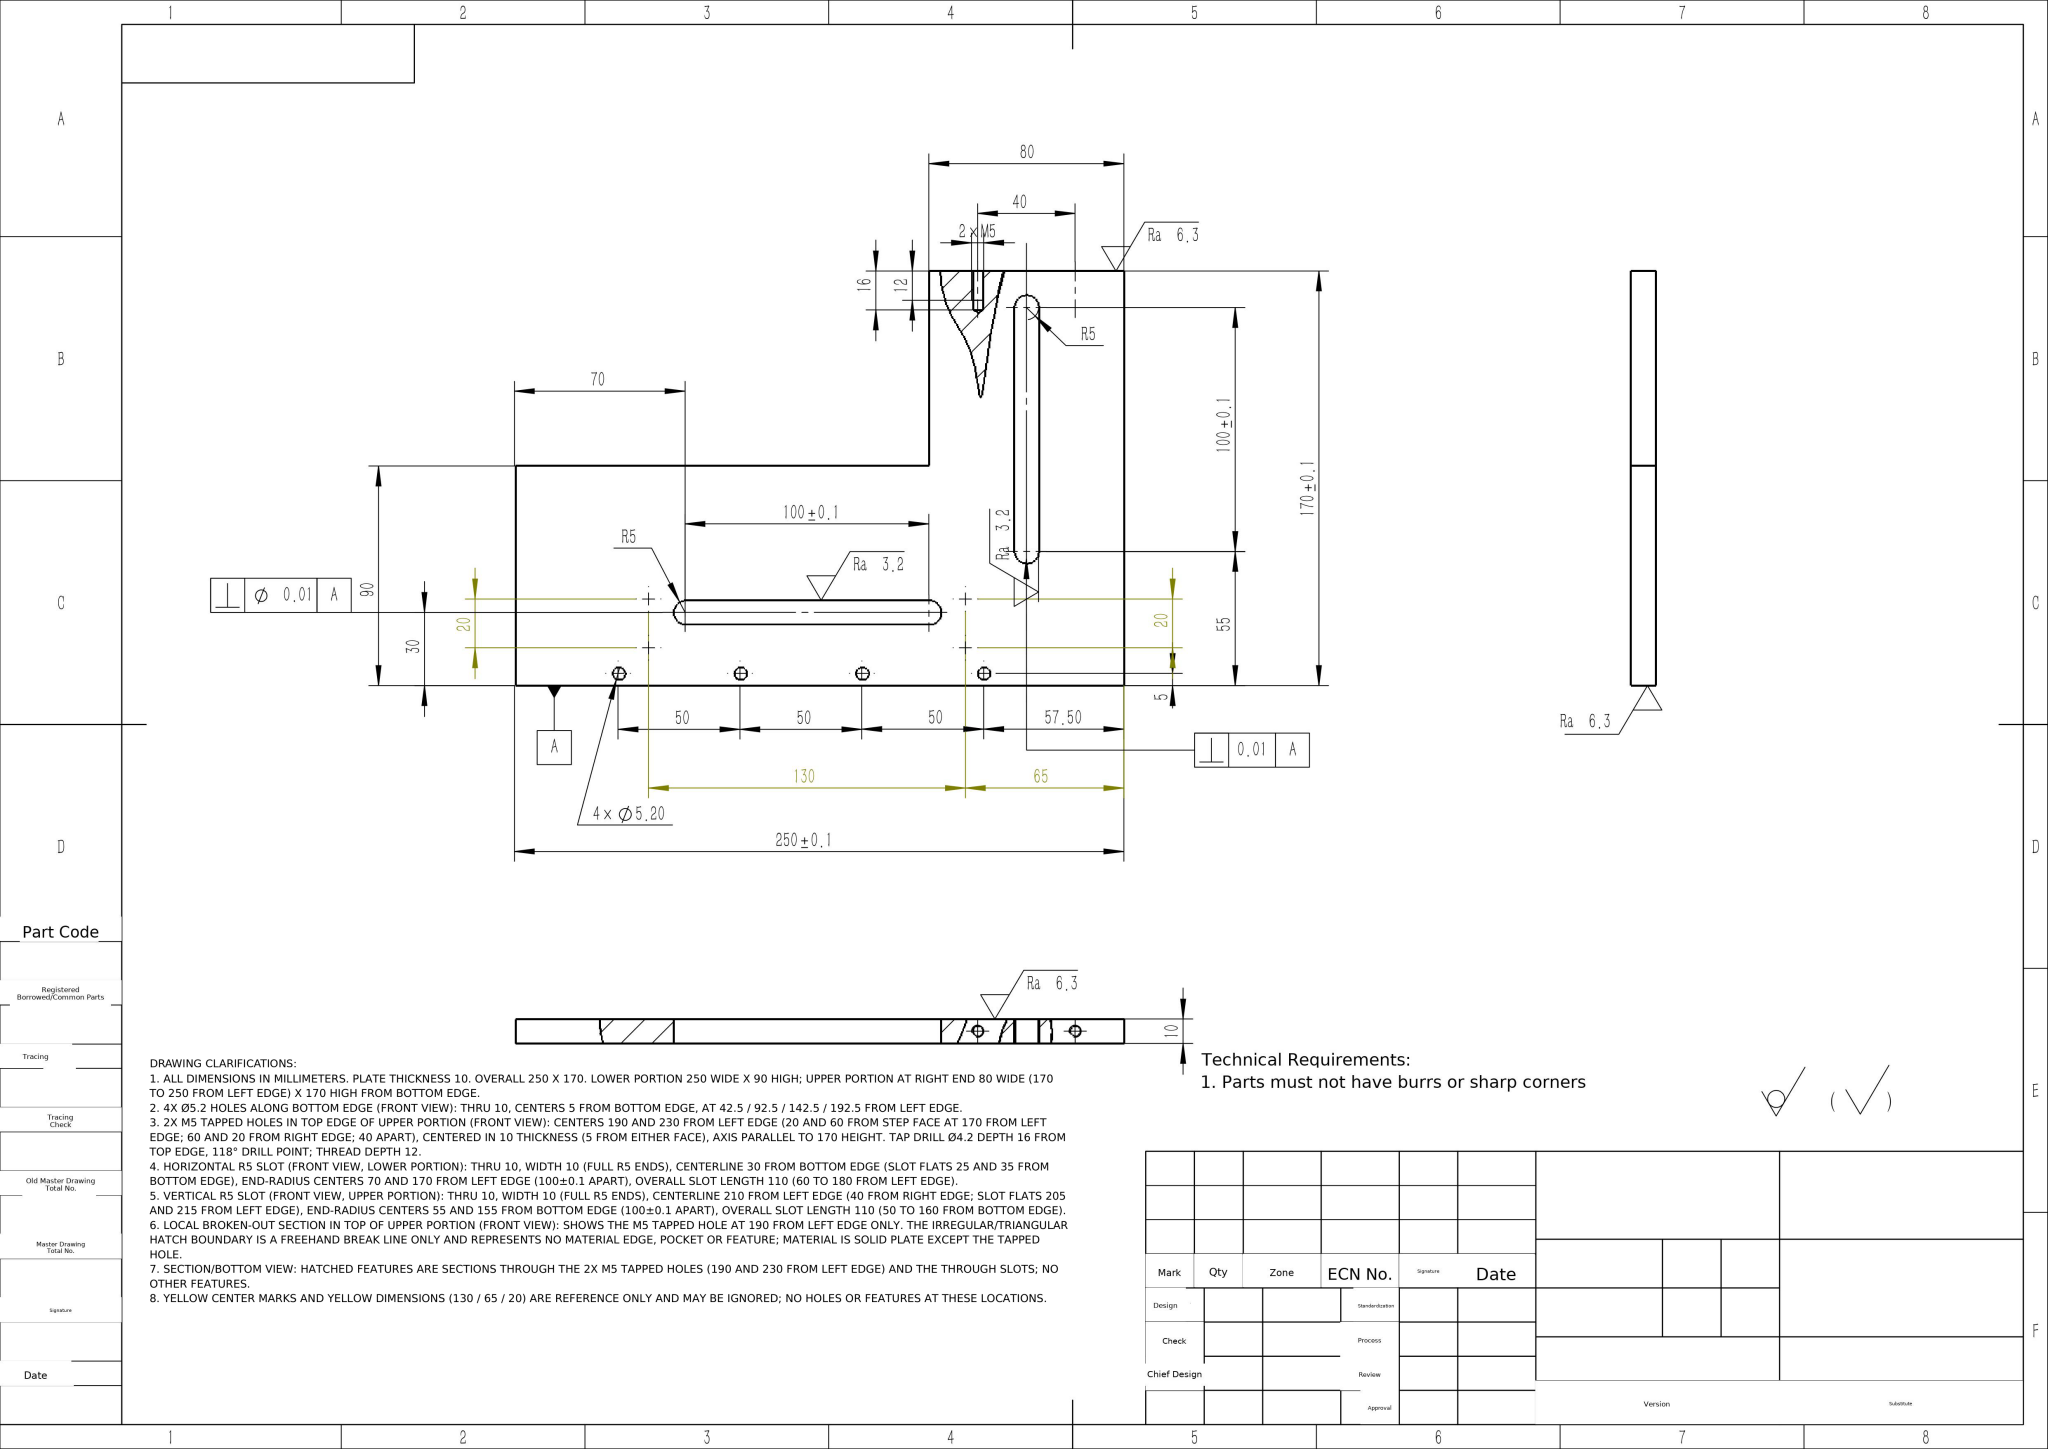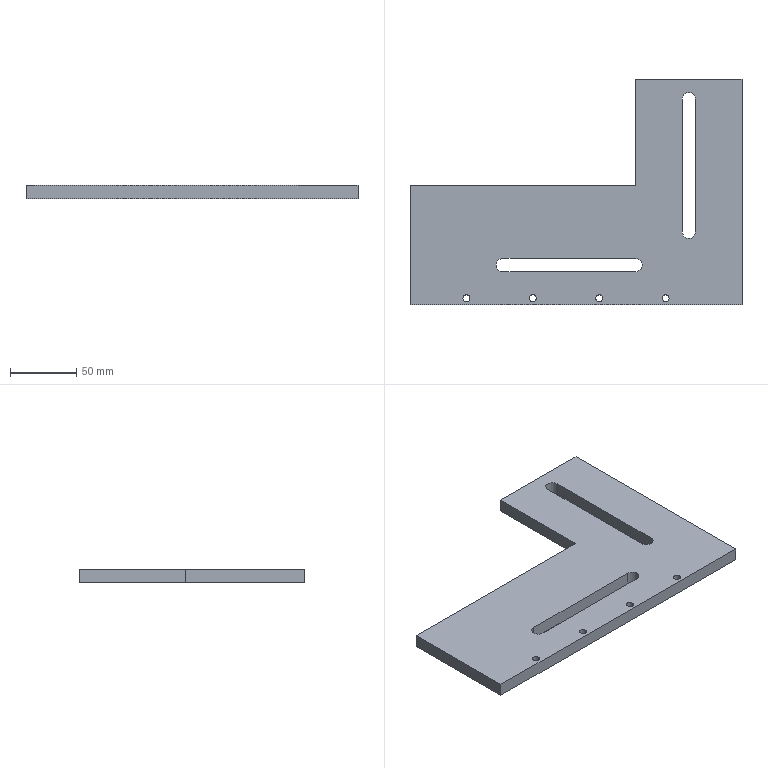Part | NX | mm | 1 solid | 33 faces | box 250 x 170 x 10 mm | volume 266125 mm3 | cylinder 17 | plane 12 | cone 4 | commonest cylinder face diameters 5.2 x8 10 x5 4.2 x4